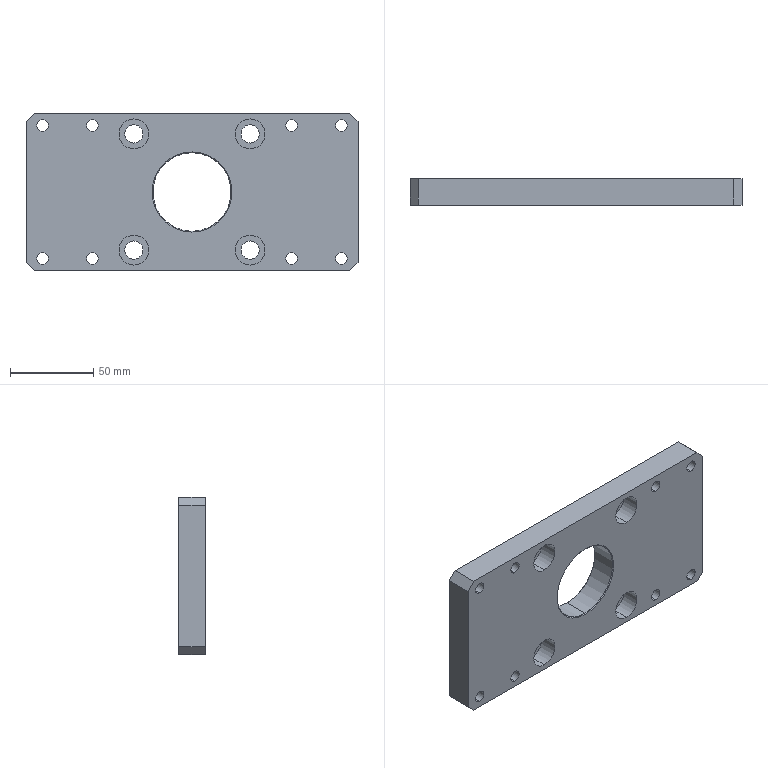Component | SolidWorks | E001CylinderRearFlangePlate-1 | 1 solid | 52 faces | box 200 x 16 x 95 mm | volume 257025 mm3 | cylinder 34 | plane 14 | cone 4 | commonest cylinder face diameters 7 x16 18 x8 11 x8 47.3 x2 | material Plain Carbon Steel
build123d program:
from build123d import *

# Parameters (mm, degrees)
SKETCH1_W                                            = 95
SKETCH1_H                                            = 200
BOSS_EXTRUDE1_DEPTH                                  = 16
HOLE_SIZE_ACCORDING_TO_THE_TYPE_OF_HEXAG_D           = 11
HOLE_SIZE_ACCORDING_TO_THE_TYPE_OF_HEXAG_CBORE_D     = 18
HOLE_SIZE_ACCORDING_TO_THE_TYPE_OF_HEXAG_CBORE_DEPTH = 11
CIRPATTERN1_COUNT                                    = 4
CHAMFER1_SIZE                                        = 5
SKETCH5_R                                            = 3.5
CUT_EXTRUDE1_DEPTH                                   = 112.858
LPATTERN1_COUNT                                      = 2
LPATTERN1_PITCH                                      = 80
LPATTERN1_COUNT_DIR2                                 = 2
LPATTERN1_PITCH_DIR2                                 = 30
MIRROR1_COPY_1_SKETCH_R                              = 3.5
MIRROR1_COPY_1_DEPTH                                 = 112.858
MIRROR1_COPY_2_SKETCH_R                              = 3.5
MIRROR1_COPY_2_DEPTH                                 = 112.858
MIRROR1_COPY_3_SKETCH_R                              = 3.5
MIRROR1_COPY_3_DEPTH                                 = 112.858


with BuildPart() as part:
    # Sketch1 → Boss-Extrude1 (new body)
    with BuildSketch(Plane(origin=(0, 0, 0), x_dir=(0, 0, -1), z_dir=(1, 0, 0))):
        Rectangle(SKETCH1_W, SKETCH1_H)
    extrude(amount=BOSS_EXTRUDE1_DEPTH)

    # Sketch2 → Cut-Revolve1 (revolve, cut)
    with BuildSketch(Plane(origin=(0, 0, 0), x_dir=(1, 0, 0), z_dir=(0, 1, 0))):
        Polygon((16, 0), (16, -24.15), (15.5, -23.65), (0.5, -23.65), (0, -24.15), (0, 0), align=None)
    revolve(axis=Axis((0, 0, 0), (1, 0, 0)), mode=Mode.SUBTRACT)

    # Hole Size according to the type of Hexag (through all)
    with Locations(Plane.ZY):
        with Locations((35, 35)):
            hole_size_according_to_the_type_of_hexag = CounterBoreHole(HOLE_SIZE_ACCORDING_TO_THE_TYPE_OF_HEXAG_D / 2, HOLE_SIZE_ACCORDING_TO_THE_TYPE_OF_HEXAG_CBORE_D / 2, HOLE_SIZE_ACCORDING_TO_THE_TYPE_OF_HEXAG_CBORE_DEPTH)

    # CirPattern1: Hole Size according to the type of Hexag ×4 about axis
    cirpattern1_axis = Axis((0, 0, 0), (1, 0, 0))
    for i in range(1, CIRPATTERN1_COUNT):
        add(hole_size_according_to_the_type_of_hexag.rotate(cirpattern1_axis, i * 360 / CIRPATTERN1_COUNT), mode=Mode.SUBTRACT)

    # Chamfer1
    chamfer1_edges = [part.edges().sort_by_distance(p)[0] for p in [
        (8, -100, -47.5),
        (8, -100, 47.5),
        (8, 100, 47.5),
        (8, 100, -47.5),
    ]]
    chamfer(chamfer1_edges, length=CHAMFER1_SIZE)

    # Sketch5 → Cut-Extrude1 (cut, through all)
    with BuildSketch(Plane.ZY):
        with Locations((-40, 90)):
            Circle(SKETCH5_R)
    cut_extrude1 = extrude(amount=-CUT_EXTRUDE1_DEPTH, mode=Mode.SUBTRACT)

    # LPattern1: Cut-Extrude1 2 × 2
    with Locations(*[(0, -j * LPATTERN1_PITCH_DIR2, i * LPATTERN1_PITCH) for i in range(LPATTERN1_COUNT) for j in range(LPATTERN1_COUNT_DIR2) if (i, j) != (0, 0)]):
        add(cut_extrude1, mode=Mode.SUBTRACT)

    # Mirror1: Cut-Extrude1 across plane
    add(cut_extrude1.mirror(Plane.ZX), mode=Mode.SUBTRACT)

    # Mirror1 copy 1 sketch → Mirror1 copy 1 (cut, through all)
    with BuildSketch(Plane(origin=(0, 30, 0), x_dir=(0, 0, 1), z_dir=(-1, 0, 0))):
        with Locations((-40, -90)):
            Circle(MIRROR1_COPY_1_SKETCH_R)
    extrude(amount=-MIRROR1_COPY_1_DEPTH, mode=Mode.SUBTRACT)

    # Mirror1 copy 2 sketch → Mirror1 copy 2 (cut, through all)
    with BuildSketch(Plane(origin=(0, 0, 80), x_dir=(0, 0, 1), z_dir=(-1, 0, 0))):
        with Locations((-40, -90)):
            Circle(MIRROR1_COPY_2_SKETCH_R)
    extrude(amount=-MIRROR1_COPY_2_DEPTH, mode=Mode.SUBTRACT)

    # Mirror1 copy 3 sketch → Mirror1 copy 3 (cut, through all)
    with BuildSketch(Plane(origin=(0, 30, 80), x_dir=(0, 0, 1), z_dir=(-1, 0, 0))):
        with Locations((-40, -90)):
            Circle(MIRROR1_COPY_3_SKETCH_R)
    extrude(amount=-MIRROR1_COPY_3_DEPTH, mode=Mode.SUBTRACT)


solid = part.part

# Placed as in the assembly
solid = solid.moved(Location((0, 0, 0), (0, 0, 90)))